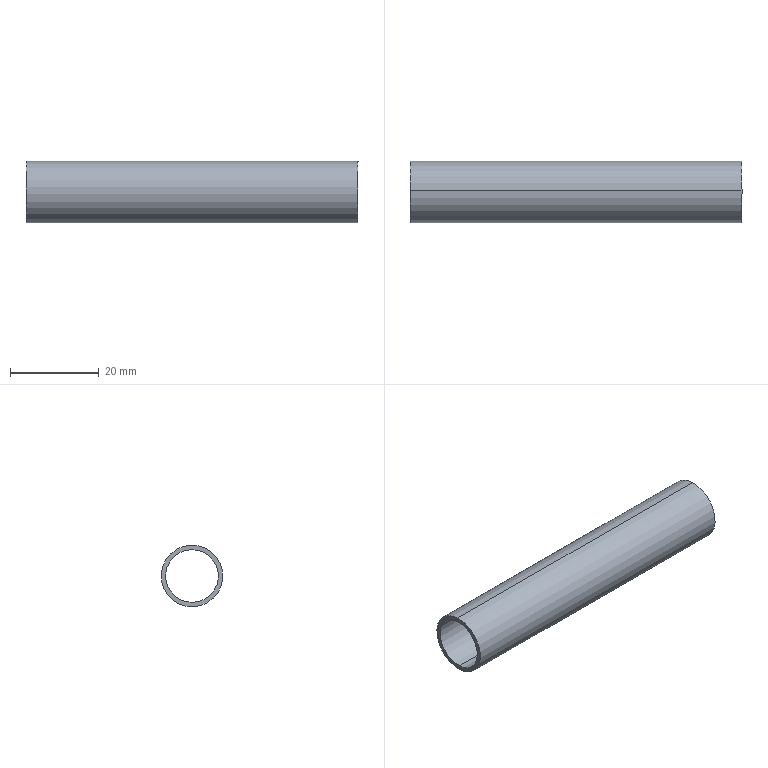Component | SolidWorks | HZ022-PenHolder1-1 | 1 solid | 6 faces | box 75 x 13.9 x 13.9 mm | volume 3039 mm3 | cylinder 4 | plane 2 | commonest cylinder face diameters 11.9 x2 13.9 x2
build123d program:
from build123d import *

# Parameters (mm, degrees)
SKETCH1_R           = 6.95
SKETCH1_R_2         = 5.95
EXTRUDE_THIN1_DEPTH = 75


with BuildPart() as part:
    # Sketch1 → Extrude-Thin1 (new body)
    with BuildSketch(Plane(origin=(0, 0, 0), x_dir=(1, 0, 0), z_dir=(0, 1, 0))):
        Circle(SKETCH1_R)
        Circle(SKETCH1_R_2, mode=Mode.SUBTRACT)
    extrude(amount=EXTRUDE_THIN1_DEPTH)


solid = part.part

# Placed as in the assembly
solid = solid.moved(Location((72.944, 126.652, 927), (0, 0, 90)))
STEP:
#1=COLOUR_RGB('',0.7922,0.8196,0.9333);
#2=FILL_AREA_STYLE_COLOUR('',#1);
#3=FILL_AREA_STYLE('',(#2));
#4=SURFACE_STYLE_FILL_AREA(#3);
#5=SURFACE_SIDE_STYLE('',(#4));
#6=SURFACE_STYLE_USAGE(.BOTH.,#5);
#7=PRESENTATION_STYLE_ASSIGNMENT((#6));
#8=CARTESIAN_POINT('',(2.872,4.976,36.262));
#9=VERTEX_POINT('',#8);
#10=CARTESIAN_POINT('',(2.872,4.997,36.73));
#11=VERTEX_POINT('',#10);
#12=CARTESIAN_POINT('',(2.872,4.986,36.496));
#13=DIRECTION('',(1.,0.,-0.));
#14=DIRECTION('',(0.,-0.999,0.045));
#15=AXIS2_PLACEMENT_3D('',#12,#13,#14);
#16=CIRCLE('',#15,0.2343);
#17=EDGE_CURVE('',#9,#11,#16,.T.);
#18=ORIENTED_EDGE('',*,*,#17,.T.);
#19=CARTESIAN_POINT('',(-0.08096,4.997,36.73));
#20=VERTEX_POINT('',#19);
#21=CARTESIAN_POINT('',(2.872,4.997,36.73));
#22=DIRECTION('',(-1.,-0.,0.));
#23=VECTOR('',#22,39.37);
#24=LINE('',#21,#23);
#25=EDGE_CURVE('',#11,#20,#24,.T.);
#26=ORIENTED_EDGE('',*,*,#25,.T.);
#27=CARTESIAN_POINT('',(-0.08096,4.976,36.262));
#28=VERTEX_POINT('',#27);
#29=CARTESIAN_POINT('',(-0.08096,4.986,36.496));
#30=DIRECTION('',(1.,0.,-0.));
#31=DIRECTION('',(0.,-0.999,0.045));
#32=AXIS2_PLACEMENT_3D('',#29,#30,#31);
#33=CIRCLE('',#32,0.2343);
#34=EDGE_CURVE('',#28,#20,#33,.T.);
#35=ORIENTED_EDGE('',*,*,#34,.F.);
#36=CARTESIAN_POINT('',(2.872,4.976,36.262));
#37=DIRECTION('',(-1.,-0.,0.));
#38=VECTOR('',#37,39.37);
#39=LINE('',#36,#38);
#40=EDGE_CURVE('',#9,#28,#39,.T.);
#41=ORIENTED_EDGE('',*,*,#40,.F.);
#42=EDGE_LOOP('',(#18,#26,#35,#41));
#43=FACE_OUTER_BOUND('',#42,.T.);
#44=CARTESIAN_POINT('',(2.872,4.986,36.496));
#45=DIRECTION('',(-1.,-0.,0.));
#46=DIRECTION('',(-0.,-0.045,-0.999));
#47=AXIS2_PLACEMENT_3D('',#44,#45,#46);
#48=CYLINDRICAL_SURFACE('',#47,0.2343);
#49=ADVANCED_FACE('',(#43),#48,.F.);
#50=CARTESIAN_POINT('',(2.872,4.999,36.769));
#51=VERTEX_POINT('',#50);
#52=CARTESIAN_POINT('',(2.872,4.974,36.223));
#53=VERTEX_POINT('',#52);
#54=CARTESIAN_POINT('',(2.872,4.986,36.496));
#55=DIRECTION('',(1.,0.,-0.));
#56=DIRECTION('',(0.,0.045,0.999));
#57=AXIS2_PLACEMENT_3D('',#54,#55,#56);
#58=CIRCLE('',#57,0.2736);
#59=EDGE_CURVE('',#51,#53,#58,.T.);
#60=ORIENTED_EDGE('',*,*,#59,.F.);
#61=CARTESIAN_POINT('',(-0.08096,4.999,36.769));
#62=VERTEX_POINT('',#61);
#63=CARTESIAN_POINT('',(2.872,4.999,36.769));
#64=DIRECTION('',(-1.,-0.,0.));
#65=VECTOR('',#64,39.37);
#66=LINE('',#63,#65);
#67=EDGE_CURVE('',#51,#62,#66,.T.);
#68=ORIENTED_EDGE('',*,*,#67,.T.);
#69=CARTESIAN_POINT('',(-0.08096,4.974,36.223));
#70=VERTEX_POINT('',#69);
#71=CARTESIAN_POINT('',(-0.08096,4.986,36.496));
#72=DIRECTION('',(1.,0.,-0.));
#73=DIRECTION('',(0.,0.045,0.999));
#74=AXIS2_PLACEMENT_3D('',#71,#72,#73);
#75=CIRCLE('',#74,0.2736);
#76=EDGE_CURVE('',#62,#70,#75,.T.);
#77=ORIENTED_EDGE('',*,*,#76,.T.);
#78=CARTESIAN_POINT('',(2.872,4.974,36.223));
#79=DIRECTION('',(-1.,-0.,0.));
#80=VECTOR('',#79,39.37);
#81=LINE('',#78,#80);
#82=EDGE_CURVE('',#53,#70,#81,.T.);
#83=ORIENTED_EDGE('',*,*,#82,.F.);
#84=EDGE_LOOP('',(#60,#68,#77,#83));
#85=FACE_OUTER_BOUND('',#84,.T.);
#86=CARTESIAN_POINT('',(2.872,4.986,36.496));
#87=DIRECTION('',(-1.,-0.,0.));
#88=DIRECTION('',(-0.,-0.045,-0.999));
#89=AXIS2_PLACEMENT_3D('',#86,#87,#88);
#90=CYLINDRICAL_SURFACE('',#89,0.2736);
#91=ADVANCED_FACE('',(#85),#90,.T.);
#92=CARTESIAN_POINT('',(2.872,4.986,36.496));
#93=DIRECTION('',(1.,0.,-0.));
#94=DIRECTION('',(0.,0.045,0.999));
#95=AXIS2_PLACEMENT_3D('',#92,#93,#94);
#96=CIRCLE('',#95,0.2736);
#97=EDGE_CURVE('',#53,#51,#96,.T.);
#98=ORIENTED_EDGE('',*,*,#97,.T.);
#99=ORIENTED_EDGE('',*,*,#59,.T.);
#100=EDGE_LOOP('',(#98,#99));
#101=FACE_OUTER_BOUND('',#100,.T.);
#102=ORIENTED_EDGE('',*,*,#17,.F.);
#103=CARTESIAN_POINT('',(2.872,4.986,36.496));
#104=DIRECTION('',(1.,0.,-0.));
#105=DIRECTION('',(0.,-0.999,0.045));
#106=AXIS2_PLACEMENT_3D('',#103,#104,#105);
#107=CIRCLE('',#106,0.2343);
#108=EDGE_CURVE('',#11,#9,#107,.T.);
#109=ORIENTED_EDGE('',*,*,#108,.F.);
#110=EDGE_LOOP('',(#102,#109));
#111=FACE_BOUND('',#110,.T.);
#112=CARTESIAN_POINT('',(2.872,4.986,36.496));
#113=DIRECTION('',(1.,0.,-0.));
#114=DIRECTION('',(0.,0.045,0.999));
#115=AXIS2_PLACEMENT_3D('',#112,#113,#114);
#116=PLANE('',#115);
#117=ADVANCED_FACE('',(#101,#111),#116,.T.);
#118=CARTESIAN_POINT('',(-0.08096,4.986,36.496));
#119=DIRECTION('',(1.,0.,-0.));
#120=DIRECTION('',(0.,0.045,0.999));
#121=AXIS2_PLACEMENT_3D('',#118,#119,#120);
#122=CIRCLE('',#121,0.2736);
#123=EDGE_CURVE('',#70,#62,#122,.T.);
#124=ORIENTED_EDGE('',*,*,#123,.F.);
#125=ORIENTED_EDGE('',*,*,#76,.F.);
#126=EDGE_LOOP('',(#124,#125));
#127=FACE_OUTER_BOUND('',#126,.T.);
#128=ORIENTED_EDGE('',*,*,#34,.T.);
#129=CARTESIAN_POINT('',(-0.08096,4.986,36.496));
#130=DIRECTION('',(1.,0.,-0.));
#131=DIRECTION('',(0.,-0.999,0.045));
#132=AXIS2_PLACEMENT_3D('',#129,#130,#131);
#133=CIRCLE('',#132,0.2343);
#134=EDGE_CURVE('',#20,#28,#133,.T.);
#135=ORIENTED_EDGE('',*,*,#134,.T.);
#136=EDGE_LOOP('',(#128,#135));
#137=FACE_BOUND('',#136,.T.);
#138=CARTESIAN_POINT('',(-0.08096,4.986,36.496));
#139=DIRECTION('',(1.,0.,-0.));
#140=DIRECTION('',(0.,0.045,0.999));
#141=AXIS2_PLACEMENT_3D('',#138,#139,#140);
#142=PLANE('',#141);
#143=ADVANCED_FACE('',(#127,#137),#142,.F.);
#144=ORIENTED_EDGE('',*,*,#67,.F.);
#145=ORIENTED_EDGE('',*,*,#97,.F.);
#146=ORIENTED_EDGE('',*,*,#82,.T.);
#147=ORIENTED_EDGE('',*,*,#123,.T.);
#148=EDGE_LOOP('',(#144,#145,#146,#147));
#149=FACE_OUTER_BOUND('',#148,.T.);
#150=CARTESIAN_POINT('',(2.872,4.986,36.496));
#151=DIRECTION('',(-1.,-0.,0.));
#152=DIRECTION('',(-0.,-0.045,-0.999));
#153=AXIS2_PLACEMENT_3D('',#150,#151,#152);
#154=CYLINDRICAL_SURFACE('',#153,0.2736);
#155=ADVANCED_FACE('',(#149),#154,.T.);
#156=ORIENTED_EDGE('',*,*,#25,.F.);
#157=ORIENTED_EDGE('',*,*,#108,.T.);
#158=ORIENTED_EDGE('',*,*,#40,.T.);
#159=ORIENTED_EDGE('',*,*,#134,.F.);
#160=EDGE_LOOP('',(#156,#157,#158,#159));
#161=FACE_OUTER_BOUND('',#160,.T.);
#162=CARTESIAN_POINT('',(2.872,4.986,36.496));
#163=DIRECTION('',(-1.,-0.,0.));
#164=DIRECTION('',(-0.,-0.045,-0.999));
#165=AXIS2_PLACEMENT_3D('',#162,#163,#164);
#166=CYLINDRICAL_SURFACE('',#165,0.2343);
#167=ADVANCED_FACE('',(#161),#166,.F.);
#168=CLOSED_SHELL('',(#49,#91,#117,#143,#155,#167));
#169=MANIFOLD_SOLID_BREP('',#168);
#170=STYLED_ITEM('',(#7),#169);
#171=(LENGTH_UNIT()NAMED_UNIT(*)SI_UNIT($,.METRE.));
#172=LENGTH_MEASURE_WITH_UNIT(LENGTH_MEASURE(0.0254),#171);
#173=DIMENSIONAL_EXPONENTS(1.,0.,0.,0.,0.,0.,0.);
#174=(CONVERSION_BASED_UNIT('',#172)LENGTH_UNIT()NAMED_UNIT(#173));
#175=UNCERTAINTY_MEASURE_WITH_UNIT(LENGTH_MEASURE(0.00001),#174,'','');
#176=(NAMED_UNIT(*)PLANE_ANGLE_UNIT()SI_UNIT($,.RADIAN.));
#177=(NAMED_UNIT(*)SI_UNIT($,.STERADIAN.)SOLID_ANGLE_UNIT());
#178=(GEOMETRIC_REPRESENTATION_CONTEXT(3)GLOBAL_UNCERTAINTY_ASSIGNED_CONTEXT((#175))GLOBAL_UNIT_ASSIGNED_CONTEXT((#174,#176,#177))REPRESENTATION_CONTEXT('',''));
#179=MECHANICAL_DESIGN_GEOMETRIC_PRESENTATION_REPRESENTATION('',(#170),#178);
#180=PRESENTATION_LAYER_ASSIGNMENT('','',(#170));
#181=CARTESIAN_POINT('',(0.,0.,0.));
#182=DIRECTION('',(0.,0.,1.));
#183=DIRECTION('',(1.,0.,0.));
#184=AXIS2_PLACEMENT_3D('',#181,#182,#183);
#185=(LENGTH_UNIT()NAMED_UNIT(*)SI_UNIT($,.METRE.));
#186=LENGTH_MEASURE_WITH_UNIT(LENGTH_MEASURE(0.0254),#185);
#187=DIMENSIONAL_EXPONENTS(1.,0.,0.,0.,0.,0.,0.);
#188=(CONVERSION_BASED_UNIT('',#186)LENGTH_UNIT()NAMED_UNIT(#187));
#189=UNCERTAINTY_MEASURE_WITH_UNIT(LENGTH_MEASURE(0.00001),#188,'','');
#190=(NAMED_UNIT(*)PLANE_ANGLE_UNIT()SI_UNIT($,.RADIAN.));
#191=(NAMED_UNIT(*)SI_UNIT($,.STERADIAN.)SOLID_ANGLE_UNIT());
#192=(GEOMETRIC_REPRESENTATION_CONTEXT(3)GLOBAL_UNCERTAINTY_ASSIGNED_CONTEXT((#189))GLOBAL_UNIT_ASSIGNED_CONTEXT((#188,#190,#191))REPRESENTATION_CONTEXT('',''));
#193=ADVANCED_BREP_SHAPE_REPRESENTATION('',(#169,#184),#192);